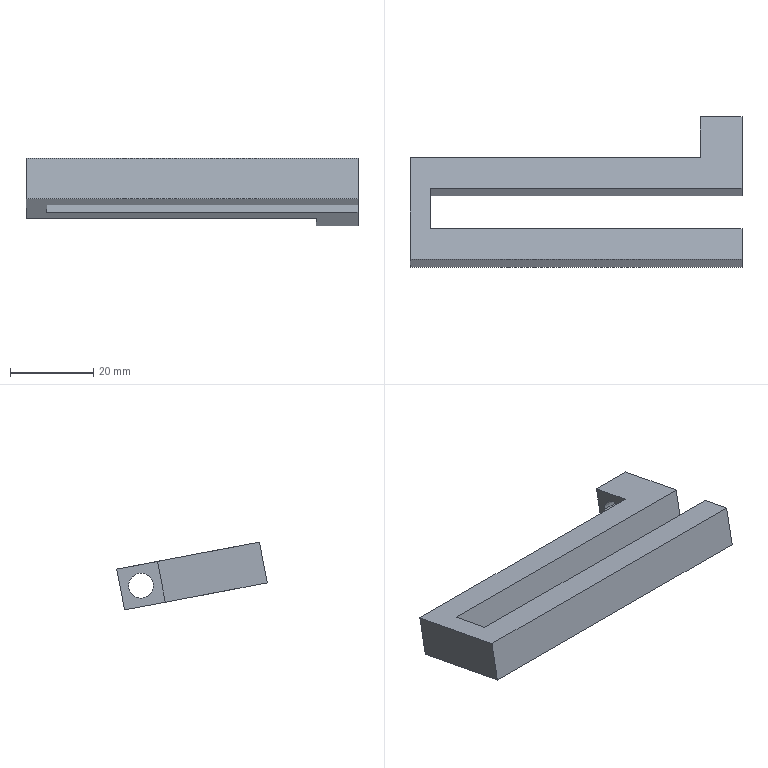Component | SolidWorks | ElectricalBoxAssembly2-1_NylonGuideBlock-1 | 1 solid | 14 faces | box 80 x 36.25 x 16.36 mm | volume 13217 mm3 | plane 12 | cylinder 2 | commonest cylinder face diameters 6 x2
build123d program:
from build123d import *

# Parameters (mm, degrees)
BOSS_EXTRUDE1_DEPTH = 10
SKETCH2_R           = 3
CUT_EXTRUDE1_DEPTH  = 83.5


with BuildPart() as part:
    # Sketch1 → Boss-Extrude1 (new body)
    with BuildSketch(Plane.XY):
        Polygon((-35.667, 17.5), (-35.667, 10), (39.333, 10), (39.333, 0), (-35.667, 0), (-35.667, -17.5), (-25.667, -17.5), (-25.667, -7.5), (44.333, -7.5), (44.333, 17.5), align=None)
    extrude(amount=BOSS_EXTRUDE1_DEPTH)

    # Sketch2 → Cut-Extrude1 (cut, through all)
    with BuildSketch(Plane.ZY.offset(35.667)):
        with Locations(Location((5, -12.5, 0), (0, 0, 270))):
            Circle(SKETCH2_R)
    extrude(amount=-CUT_EXTRUDE1_DEPTH, mode=Mode.SUBTRACT)


solid = part.part

# Placed as in the assembly
solid = solid.moved(Location((704.802, 360.896, 1985.392), (-10.755, 0, 180)))
STEP:
#1=COLOUR_RGB('',0.7922,0.8196,0.9333);
#2=FILL_AREA_STYLE_COLOUR('',#1);
#3=FILL_AREA_STYLE('',(#2));
#4=SURFACE_STYLE_FILL_AREA(#3);
#5=SURFACE_SIDE_STYLE('',(#4));
#6=SURFACE_STYLE_USAGE(.BOTH.,#5);
#7=PRESENTATION_STYLE_ASSIGNMENT((#6));
#8=CARTESIAN_POINT('',(28.759,14.613,78.289));
#9=VERTEX_POINT('',#8);
#10=CARTESIAN_POINT('',(28.759,14.845,78.245));
#11=VERTEX_POINT('',#10);
#12=CARTESIAN_POINT('',(28.759,14.729,78.267));
#13=DIRECTION('',(1.,-0.,0.));
#14=DIRECTION('',(0.,0.9824,-0.1866));
#15=AXIS2_PLACEMENT_3D('',#12,#13,#14);
#16=CIRCLE('',#15,0.1181);
#17=EDGE_CURVE('',#9,#11,#16,.T.);
#18=ORIENTED_EDGE('',*,*,#17,.F.);
#19=CARTESIAN_POINT('',(29.152,14.613,78.289));
#20=VERTEX_POINT('',#19);
#21=CARTESIAN_POINT('',(26.003,14.613,78.289));
#22=DIRECTION('',(1.,0.,0.));
#23=VECTOR('',#22,39.37);
#24=LINE('',#21,#23);
#25=EDGE_CURVE('',#9,#20,#24,.T.);
#26=ORIENTED_EDGE('',*,*,#25,.T.);
#27=CARTESIAN_POINT('',(29.152,14.845,78.245));
#28=VERTEX_POINT('',#27);
#29=CARTESIAN_POINT('',(29.152,14.729,78.267));
#30=DIRECTION('',(1.,0.,0.));
#31=DIRECTION('',(0.,0.9824,-0.1866));
#32=AXIS2_PLACEMENT_3D('',#29,#30,#31);
#33=CIRCLE('',#32,0.1181);
#34=EDGE_CURVE('',#20,#28,#33,.T.);
#35=ORIENTED_EDGE('',*,*,#34,.T.);
#36=CARTESIAN_POINT('',(26.003,14.845,78.245));
#37=DIRECTION('',(1.,0.,0.));
#38=VECTOR('',#37,39.37);
#39=LINE('',#36,#38);
#40=EDGE_CURVE('',#11,#28,#39,.T.);
#41=ORIENTED_EDGE('',*,*,#40,.F.);
#42=EDGE_LOOP('',(#18,#26,#35,#41));
#43=FACE_OUTER_BOUND('',#42,.T.);
#44=CARTESIAN_POINT('',(26.003,14.729,78.267));
#45=DIRECTION('',(1.,0.,0.));
#46=DIRECTION('',(0.,0.9824,-0.1866));
#47=AXIS2_PLACEMENT_3D('',#44,#45,#46);
#48=CYLINDRICAL_SURFACE('',#47,0.1181);
#49=ADVANCED_FACE('',(#43),#48,.F.);
#50=CARTESIAN_POINT('',(26.003,13.532,78.294));
#51=VERTEX_POINT('',#50);
#52=CARTESIAN_POINT('',(29.152,13.532,78.294));
#53=VERTEX_POINT('',#52);
#54=CARTESIAN_POINT('',(29.152,13.532,78.294));
#55=DIRECTION('',(1.,-0.,0.));
#56=VECTOR('',#55,39.37);
#57=LINE('',#54,#56);
#58=EDGE_CURVE('',#51,#53,#57,.T.);
#59=ORIENTED_EDGE('',*,*,#58,.T.);
#60=CARTESIAN_POINT('',(29.152,13.605,78.68));
#61=VERTEX_POINT('',#60);
#62=CARTESIAN_POINT('',(29.152,13.605,78.68));
#63=DIRECTION('',(0.,-0.1866,-0.9824));
#64=VECTOR('',#63,39.37);
#65=LINE('',#62,#64);
#66=EDGE_CURVE('',#61,#53,#65,.T.);
#67=ORIENTED_EDGE('',*,*,#66,.F.);
#68=CARTESIAN_POINT('',(26.003,13.605,78.68));
#69=VERTEX_POINT('',#68);
#70=CARTESIAN_POINT('',(29.152,13.605,78.68));
#71=DIRECTION('',(1.,-0.,0.));
#72=VECTOR('',#71,39.37);
#73=LINE('',#70,#72);
#74=EDGE_CURVE('',#69,#61,#73,.T.);
#75=ORIENTED_EDGE('',*,*,#74,.F.);
#76=CARTESIAN_POINT('',(26.003,13.605,78.68));
#77=DIRECTION('',(0.,-0.1866,-0.9824));
#78=VECTOR('',#77,39.37);
#79=LINE('',#76,#78);
#80=EDGE_CURVE('',#69,#51,#79,.T.);
#81=ORIENTED_EDGE('',*,*,#80,.T.);
#82=EDGE_LOOP('',(#59,#67,#75,#81));
#83=FACE_OUTER_BOUND('',#82,.T.);
#84=CARTESIAN_POINT('',(29.152,13.605,78.68));
#85=DIRECTION('',(0.,0.9824,-0.1866));
#86=DIRECTION('',(-1.,0.,-0.));
#87=AXIS2_PLACEMENT_3D('',#84,#85,#86);
#88=PLANE('',#87);
#89=ADVANCED_FACE('',(#83),#88,.F.);
#90=CARTESIAN_POINT('',(29.152,13.822,78.239));
#91=VERTEX_POINT('',#90);
#92=CARTESIAN_POINT('',(29.152,13.532,78.294));
#93=DIRECTION('',(0.,0.9824,-0.1866));
#94=VECTOR('',#93,39.37);
#95=LINE('',#92,#94);
#96=EDGE_CURVE('',#53,#91,#95,.T.);
#97=ORIENTED_EDGE('',*,*,#96,.T.);
#98=CARTESIAN_POINT('',(29.152,13.895,78.625));
#99=VERTEX_POINT('',#98);
#100=CARTESIAN_POINT('',(29.152,13.895,78.625));
#101=DIRECTION('',(0.,-0.1866,-0.9824));
#102=VECTOR('',#101,39.37);
#103=LINE('',#100,#102);
#104=EDGE_CURVE('',#99,#91,#103,.T.);
#105=ORIENTED_EDGE('',*,*,#104,.F.);
#106=CARTESIAN_POINT('',(29.152,13.605,78.68));
#107=DIRECTION('',(0.,0.9824,-0.1866));
#108=VECTOR('',#107,39.37);
#109=LINE('',#106,#108);
#110=EDGE_CURVE('',#61,#99,#109,.T.);
#111=ORIENTED_EDGE('',*,*,#110,.F.);
#112=ORIENTED_EDGE('',*,*,#66,.T.);
#113=EDGE_LOOP('',(#97,#105,#111,#112));
#114=FACE_OUTER_BOUND('',#113,.T.);
#115=CARTESIAN_POINT('',(29.152,13.605,78.68));
#116=DIRECTION('',(-1.,0.,-0.));
#117=DIRECTION('',(0.,-0.1866,-0.9824));
#118=AXIS2_PLACEMENT_3D('',#115,#116,#117);
#119=PLANE('',#118);
#120=ADVANCED_FACE('',(#114),#119,.F.);
#121=CARTESIAN_POINT('',(26.2,13.822,78.239));
#122=VERTEX_POINT('',#121);
#123=CARTESIAN_POINT('',(29.152,13.822,78.239));
#124=DIRECTION('',(-1.,0.,-0.));
#125=VECTOR('',#124,39.37);
#126=LINE('',#123,#125);
#127=EDGE_CURVE('',#91,#122,#126,.T.);
#128=ORIENTED_EDGE('',*,*,#127,.T.);
#129=CARTESIAN_POINT('',(26.2,13.895,78.625));
#130=VERTEX_POINT('',#129);
#131=CARTESIAN_POINT('',(26.2,13.895,78.625));
#132=DIRECTION('',(0.,-0.1866,-0.9824));
#133=VECTOR('',#132,39.37);
#134=LINE('',#131,#133);
#135=EDGE_CURVE('',#130,#122,#134,.T.);
#136=ORIENTED_EDGE('',*,*,#135,.F.);
#137=CARTESIAN_POINT('',(29.152,13.895,78.625));
#138=DIRECTION('',(-1.,0.,-0.));
#139=VECTOR('',#138,39.37);
#140=LINE('',#137,#139);
#141=EDGE_CURVE('',#99,#130,#140,.T.);
#142=ORIENTED_EDGE('',*,*,#141,.F.);
#143=ORIENTED_EDGE('',*,*,#104,.T.);
#144=EDGE_LOOP('',(#128,#136,#142,#143));
#145=FACE_OUTER_BOUND('',#144,.T.);
#146=CARTESIAN_POINT('',(29.152,13.895,78.625));
#147=DIRECTION('',(-0.,-0.9824,0.1866));
#148=DIRECTION('',(-0.,0.1866,0.9824));
#149=AXIS2_PLACEMENT_3D('',#146,#147,#148);
#150=PLANE('',#149);
#151=ADVANCED_FACE('',(#145),#150,.F.);
#152=CARTESIAN_POINT('',(26.2,14.209,78.165));
#153=VERTEX_POINT('',#152);
#154=CARTESIAN_POINT('',(26.2,13.822,78.239));
#155=DIRECTION('',(0.,0.9824,-0.1866));
#156=VECTOR('',#155,39.37);
#157=LINE('',#154,#156);
#158=EDGE_CURVE('',#122,#153,#157,.T.);
#159=ORIENTED_EDGE('',*,*,#158,.T.);
#160=CARTESIAN_POINT('',(26.2,14.282,78.552));
#161=VERTEX_POINT('',#160);
#162=CARTESIAN_POINT('',(26.2,14.282,78.552));
#163=DIRECTION('',(0.,-0.1866,-0.9824));
#164=VECTOR('',#163,39.37);
#165=LINE('',#162,#164);
#166=EDGE_CURVE('',#161,#153,#165,.T.);
#167=ORIENTED_EDGE('',*,*,#166,.F.);
#168=CARTESIAN_POINT('',(26.2,13.895,78.625));
#169=DIRECTION('',(0.,0.9824,-0.1866));
#170=VECTOR('',#169,39.37);
#171=LINE('',#168,#170);
#172=EDGE_CURVE('',#130,#161,#171,.T.);
#173=ORIENTED_EDGE('',*,*,#172,.F.);
#174=ORIENTED_EDGE('',*,*,#135,.T.);
#175=EDGE_LOOP('',(#159,#167,#173,#174));
#176=FACE_OUTER_BOUND('',#175,.T.);
#177=CARTESIAN_POINT('',(26.2,13.895,78.625));
#178=DIRECTION('',(-1.,0.,-0.));
#179=DIRECTION('',(-0.,-0.9824,0.1866));
#180=AXIS2_PLACEMENT_3D('',#177,#178,#179);
#181=PLANE('',#180);
#182=ADVANCED_FACE('',(#176),#181,.F.);
#183=CARTESIAN_POINT('',(29.152,14.209,78.165));
#184=VERTEX_POINT('',#183);
#185=CARTESIAN_POINT('',(26.2,14.209,78.165));
#186=DIRECTION('',(1.,-0.,0.));
#187=VECTOR('',#186,39.37);
#188=LINE('',#185,#187);
#189=EDGE_CURVE('',#153,#184,#188,.T.);
#190=ORIENTED_EDGE('',*,*,#189,.T.);
#191=CARTESIAN_POINT('',(29.152,14.282,78.552));
#192=VERTEX_POINT('',#191);
#193=CARTESIAN_POINT('',(29.152,14.282,78.552));
#194=DIRECTION('',(0.,-0.1866,-0.9824));
#195=VECTOR('',#194,39.37);
#196=LINE('',#193,#195);
#197=EDGE_CURVE('',#192,#184,#196,.T.);
#198=ORIENTED_EDGE('',*,*,#197,.F.);
#199=CARTESIAN_POINT('',(26.2,14.282,78.552));
#200=DIRECTION('',(1.,-0.,0.));
#201=VECTOR('',#200,39.37);
#202=LINE('',#199,#201);
#203=EDGE_CURVE('',#161,#192,#202,.T.);
#204=ORIENTED_EDGE('',*,*,#203,.F.);
#205=ORIENTED_EDGE('',*,*,#166,.T.);
#206=EDGE_LOOP('',(#190,#198,#204,#205));
#207=FACE_OUTER_BOUND('',#206,.T.);
#208=CARTESIAN_POINT('',(26.2,14.282,78.552));
#209=DIRECTION('',(0.,0.9824,-0.1866));
#210=DIRECTION('',(-1.,0.,-0.));
#211=AXIS2_PLACEMENT_3D('',#208,#209,#210);
#212=PLANE('',#211);
#213=ADVANCED_FACE('',(#207),#212,.F.);
#214=CARTESIAN_POINT('',(29.152,14.729,78.267));
#215=DIRECTION('',(1.,0.,0.));
#216=DIRECTION('',(0.,0.9824,-0.1866));
#217=AXIS2_PLACEMENT_3D('',#214,#215,#216);
#218=CIRCLE('',#217,0.1181);
#219=EDGE_CURVE('',#28,#20,#218,.T.);
#220=ORIENTED_EDGE('',*,*,#219,.F.);
#221=ORIENTED_EDGE('',*,*,#34,.F.);
#222=EDGE_LOOP('',(#220,#221));
#223=FACE_BOUND('',#222,.T.);
#224=CARTESIAN_POINT('',(29.152,14.885,78.036));
#225=VERTEX_POINT('',#224);
#226=CARTESIAN_POINT('',(29.152,14.209,78.165));
#227=DIRECTION('',(0.,0.9824,-0.1866));
#228=VECTOR('',#227,39.37);
#229=LINE('',#226,#228);
#230=EDGE_CURVE('',#184,#225,#229,.T.);
#231=ORIENTED_EDGE('',*,*,#230,.T.);
#232=CARTESIAN_POINT('',(29.152,14.959,78.423));
#233=VERTEX_POINT('',#232);
#234=CARTESIAN_POINT('',(29.152,14.959,78.423));
#235=DIRECTION('',(0.,-0.1866,-0.9824));
#236=VECTOR('',#235,39.37);
#237=LINE('',#234,#236);
#238=EDGE_CURVE('',#233,#225,#237,.T.);
#239=ORIENTED_EDGE('',*,*,#238,.F.);
#240=CARTESIAN_POINT('',(29.152,14.282,78.552));
#241=DIRECTION('',(0.,0.9824,-0.1866));
#242=VECTOR('',#241,39.37);
#243=LINE('',#240,#242);
#244=EDGE_CURVE('',#192,#233,#243,.T.);
#245=ORIENTED_EDGE('',*,*,#244,.F.);
#246=ORIENTED_EDGE('',*,*,#197,.T.);
#247=EDGE_LOOP('',(#231,#239,#245,#246));
#248=FACE_OUTER_BOUND('',#247,.T.);
#249=CARTESIAN_POINT('',(29.152,14.282,78.552));
#250=DIRECTION('',(-1.,-0.,-0.));
#251=DIRECTION('',(-0.,-0.9824,0.1866));
#252=AXIS2_PLACEMENT_3D('',#249,#250,#251);
#253=PLANE('',#252);
#254=ADVANCED_FACE('',(#223,#248),#253,.F.);
#255=CARTESIAN_POINT('',(28.759,14.885,78.036));
#256=VERTEX_POINT('',#255);
#257=CARTESIAN_POINT('',(29.152,14.885,78.036));
#258=DIRECTION('',(-1.,0.,-0.));
#259=VECTOR('',#258,39.37);
#260=LINE('',#257,#259);
#261=EDGE_CURVE('',#225,#256,#260,.T.);
#262=ORIENTED_EDGE('',*,*,#261,.T.);
#263=CARTESIAN_POINT('',(28.759,14.959,78.423));
#264=VERTEX_POINT('',#263);
#265=CARTESIAN_POINT('',(28.759,14.959,78.423));
#266=DIRECTION('',(0.,-0.1866,-0.9824));
#267=VECTOR('',#266,39.37);
#268=LINE('',#265,#267);
#269=EDGE_CURVE('',#264,#256,#268,.T.);
#270=ORIENTED_EDGE('',*,*,#269,.F.);
#271=CARTESIAN_POINT('',(29.152,14.959,78.423));
#272=DIRECTION('',(-1.,0.,-0.));
#273=VECTOR('',#272,39.37);
#274=LINE('',#271,#273);
#275=EDGE_CURVE('',#233,#264,#274,.T.);
#276=ORIENTED_EDGE('',*,*,#275,.F.);
#277=ORIENTED_EDGE('',*,*,#238,.T.);
#278=EDGE_LOOP('',(#262,#270,#276,#277));
#279=FACE_OUTER_BOUND('',#278,.T.);
#280=CARTESIAN_POINT('',(29.152,14.959,78.423));
#281=DIRECTION('',(-0.,-0.9824,0.1866));
#282=DIRECTION('',(-0.,0.1866,0.9824));
#283=AXIS2_PLACEMENT_3D('',#280,#281,#282);
#284=PLANE('',#283);
#285=ADVANCED_FACE('',(#279),#284,.F.);
#286=CARTESIAN_POINT('',(28.759,14.729,78.267));
#287=DIRECTION('',(1.,-0.,0.));
#288=DIRECTION('',(0.,0.9824,-0.1866));
#289=AXIS2_PLACEMENT_3D('',#286,#287,#288);
#290=CIRCLE('',#289,0.1181);
#291=EDGE_CURVE('',#11,#9,#290,.T.);
#292=ORIENTED_EDGE('',*,*,#291,.T.);
#293=ORIENTED_EDGE('',*,*,#17,.T.);
#294=EDGE_LOOP('',(#292,#293));
#295=FACE_BOUND('',#294,.T.);
#296=CARTESIAN_POINT('',(28.759,14.499,78.11));
#297=VERTEX_POINT('',#296);
#298=CARTESIAN_POINT('',(28.759,14.499,78.11));
#299=DIRECTION('',(-0.,-0.9824,0.1866));
#300=VECTOR('',#299,39.37);
#301=LINE('',#298,#300);
#302=EDGE_CURVE('',#256,#297,#301,.T.);
#303=ORIENTED_EDGE('',*,*,#302,.T.);
#304=CARTESIAN_POINT('',(28.759,14.572,78.497));
#305=VERTEX_POINT('',#304);
#306=CARTESIAN_POINT('',(28.759,14.572,78.497));
#307=DIRECTION('',(0.,-0.1866,-0.9824));
#308=VECTOR('',#307,39.37);
#309=LINE('',#306,#308);
#310=EDGE_CURVE('',#305,#297,#309,.T.);
#311=ORIENTED_EDGE('',*,*,#310,.F.);
#312=CARTESIAN_POINT('',(28.759,14.572,78.497));
#313=DIRECTION('',(-0.,-0.9824,0.1866));
#314=VECTOR('',#313,39.37);
#315=LINE('',#312,#314);
#316=EDGE_CURVE('',#264,#305,#315,.T.);
#317=ORIENTED_EDGE('',*,*,#316,.F.);
#318=ORIENTED_EDGE('',*,*,#269,.T.);
#319=EDGE_LOOP('',(#303,#311,#317,#318));
#320=FACE_OUTER_BOUND('',#319,.T.);
#321=CARTESIAN_POINT('',(28.759,14.572,78.497));
#322=DIRECTION('',(1.,-0.,0.));
#323=DIRECTION('',(0.,0.9824,-0.1866));
#324=AXIS2_PLACEMENT_3D('',#321,#322,#323);
#325=PLANE('',#324);
#326=ADVANCED_FACE('',(#295,#320),#325,.F.);
#327=CARTESIAN_POINT('',(26.003,14.499,78.11));
#328=VERTEX_POINT('',#327);
#329=CARTESIAN_POINT('',(26.003,14.499,78.11));
#330=DIRECTION('',(-1.,0.,-0.));
#331=VECTOR('',#330,39.37);
#332=LINE('',#329,#331);
#333=EDGE_CURVE('',#297,#328,#332,.T.);
#334=ORIENTED_EDGE('',*,*,#333,.T.);
#335=CARTESIAN_POINT('',(26.003,14.572,78.497));
#336=VERTEX_POINT('',#335);
#337=CARTESIAN_POINT('',(26.003,14.572,78.497));
#338=DIRECTION('',(0.,-0.1866,-0.9824));
#339=VECTOR('',#338,39.37);
#340=LINE('',#337,#339);
#341=EDGE_CURVE('',#336,#328,#340,.T.);
#342=ORIENTED_EDGE('',*,*,#341,.F.);
#343=CARTESIAN_POINT('',(26.003,14.572,78.497));
#344=DIRECTION('',(-1.,0.,-0.));
#345=VECTOR('',#344,39.37);
#346=LINE('',#343,#345);
#347=EDGE_CURVE('',#305,#336,#346,.T.);
#348=ORIENTED_EDGE('',*,*,#347,.F.);
#349=ORIENTED_EDGE('',*,*,#310,.T.);
#350=EDGE_LOOP('',(#334,#342,#348,#349));
#351=FACE_OUTER_BOUND('',#350,.T.);
#352=CARTESIAN_POINT('',(26.003,14.572,78.497));
#353=DIRECTION('',(-0.,-0.9824,0.1866));
#354=DIRECTION('',(1.,-0.,0.));
#355=AXIS2_PLACEMENT_3D('',#352,#353,#354);
#356=PLANE('',#355);
#357=ADVANCED_FACE('',(#351),#356,.F.);
#358=CARTESIAN_POINT('',(26.003,13.532,78.294));
#359=DIRECTION('',(-0.,-0.9824,0.1866));
#360=VECTOR('',#359,39.37);
#361=LINE('',#358,#360);
#362=EDGE_CURVE('',#328,#51,#361,.T.);
#363=ORIENTED_EDGE('',*,*,#362,.T.);
#364=ORIENTED_EDGE('',*,*,#80,.F.);
#365=CARTESIAN_POINT('',(26.003,13.605,78.68));
#366=DIRECTION('',(-0.,-0.9824,0.1866));
#367=VECTOR('',#366,39.37);
#368=LINE('',#365,#367);
#369=EDGE_CURVE('',#336,#69,#368,.T.);
#370=ORIENTED_EDGE('',*,*,#369,.F.);
#371=ORIENTED_EDGE('',*,*,#341,.T.);
#372=EDGE_LOOP('',(#363,#364,#370,#371));
#373=FACE_OUTER_BOUND('',#372,.T.);
#374=CARTESIAN_POINT('',(26.003,13.605,78.68));
#375=DIRECTION('',(1.,-0.,0.));
#376=DIRECTION('',(-0.,0.1866,0.9824));
#377=AXIS2_PLACEMENT_3D('',#374,#375,#376);
#378=PLANE('',#377);
#379=ADVANCED_FACE('',(#373),#378,.F.);
#380=ORIENTED_EDGE('',*,*,#74,.T.);
#381=ORIENTED_EDGE('',*,*,#110,.T.);
#382=ORIENTED_EDGE('',*,*,#141,.T.);
#383=ORIENTED_EDGE('',*,*,#172,.T.);
#384=ORIENTED_EDGE('',*,*,#203,.T.);
#385=ORIENTED_EDGE('',*,*,#244,.T.);
#386=ORIENTED_EDGE('',*,*,#275,.T.);
#387=ORIENTED_EDGE('',*,*,#316,.T.);
#388=ORIENTED_EDGE('',*,*,#347,.T.);
#389=ORIENTED_EDGE('',*,*,#369,.T.);
#390=EDGE_LOOP('',(#380,#381,#382,#383,#384,#385,#386,#387,#388,#389));
#391=FACE_OUTER_BOUND('',#390,.T.);
#392=CARTESIAN_POINT('',(27.748,14.282,78.552));
#393=DIRECTION('',(0.,-0.1866,-0.9824));
#394=DIRECTION('',(1.,-0.,0.));
#395=AXIS2_PLACEMENT_3D('',#392,#393,#394);
#396=PLANE('',#395);
#397=ADVANCED_FACE('',(#391),#396,.F.);
#398=ORIENTED_EDGE('',*,*,#58,.F.);
#399=ORIENTED_EDGE('',*,*,#362,.F.);
#400=ORIENTED_EDGE('',*,*,#333,.F.);
#401=ORIENTED_EDGE('',*,*,#302,.F.);
#402=ORIENTED_EDGE('',*,*,#261,.F.);
#403=ORIENTED_EDGE('',*,*,#230,.F.);
#404=ORIENTED_EDGE('',*,*,#189,.F.);
#405=ORIENTED_EDGE('',*,*,#158,.F.);
#406=ORIENTED_EDGE('',*,*,#127,.F.);
#407=ORIENTED_EDGE('',*,*,#96,.F.);
#408=EDGE_LOOP('',(#398,#399,#400,#401,#402,#403,#404,#405,#406,#407));
#409=FACE_OUTER_BOUND('',#408,.T.);
#410=CARTESIAN_POINT('',(27.748,14.209,78.165));
#411=DIRECTION('',(0.,-0.1866,-0.9824));
#412=DIRECTION('',(1.,-0.,0.));
#413=AXIS2_PLACEMENT_3D('',#410,#411,#412);
#414=PLANE('',#413);
#415=ADVANCED_FACE('',(#409),#414,.T.);
#416=ORIENTED_EDGE('',*,*,#25,.F.);
#417=ORIENTED_EDGE('',*,*,#291,.F.);
#418=ORIENTED_EDGE('',*,*,#40,.T.);
#419=ORIENTED_EDGE('',*,*,#219,.T.);
#420=EDGE_LOOP('',(#416,#417,#418,#419));
#421=FACE_OUTER_BOUND('',#420,.T.);
#422=CARTESIAN_POINT('',(26.003,14.729,78.267));
#423=DIRECTION('',(1.,0.,0.));
#424=DIRECTION('',(0.,0.9824,-0.1866));
#425=AXIS2_PLACEMENT_3D('',#422,#423,#424);
#426=CYLINDRICAL_SURFACE('',#425,0.1181);
#427=ADVANCED_FACE('',(#421),#426,.F.);
#428=CLOSED_SHELL('',(#49,#89,#120,#151,#182,#213,#254,#285,#326,#357,#379,#397,#415,#427));
#429=MANIFOLD_SOLID_BREP('',#428);
#430=STYLED_ITEM('',(#7),#429);
#431=PRESENTATION_LAYER_ASSIGNMENT('','',(#430));
#432=(LENGTH_UNIT()NAMED_UNIT(*)SI_UNIT($,.METRE.));
#433=LENGTH_MEASURE_WITH_UNIT(LENGTH_MEASURE(0.0254),#432);
#434=DIMENSIONAL_EXPONENTS(1.,0.,0.,0.,0.,0.,0.);
#435=(CONVERSION_BASED_UNIT('',#433)LENGTH_UNIT()NAMED_UNIT(#434));
#436=UNCERTAINTY_MEASURE_WITH_UNIT(LENGTH_MEASURE(0.00001),#435,'','');
#437=(NAMED_UNIT(*)PLANE_ANGLE_UNIT()SI_UNIT($,.RADIAN.));
#438=(NAMED_UNIT(*)SI_UNIT($,.STERADIAN.)SOLID_ANGLE_UNIT());
#439=(GEOMETRIC_REPRESENTATION_CONTEXT(3)GLOBAL_UNCERTAINTY_ASSIGNED_CONTEXT((#436))GLOBAL_UNIT_ASSIGNED_CONTEXT((#435,#437,#438))REPRESENTATION_CONTEXT('',''));
#440=MECHANICAL_DESIGN_GEOMETRIC_PRESENTATION_REPRESENTATION('',(#430),#439);
#441=CARTESIAN_POINT('',(0.,0.,0.));
#442=DIRECTION('',(0.,0.,1.));
#443=DIRECTION('',(1.,0.,0.));
#444=AXIS2_PLACEMENT_3D('',#441,#442,#443);
#445=(LENGTH_UNIT()NAMED_UNIT(*)SI_UNIT($,.METRE.));
#446=LENGTH_MEASURE_WITH_UNIT(LENGTH_MEASURE(0.0254),#445);
#447=DIMENSIONAL_EXPONENTS(1.,0.,0.,0.,0.,0.,0.);
#448=(CONVERSION_BASED_UNIT('',#446)LENGTH_UNIT()NAMED_UNIT(#447));
#449=UNCERTAINTY_MEASURE_WITH_UNIT(LENGTH_MEASURE(0.00001),#448,'','');
#450=(NAMED_UNIT(*)PLANE_ANGLE_UNIT()SI_UNIT($,.RADIAN.));
#451=(NAMED_UNIT(*)SI_UNIT($,.STERADIAN.)SOLID_ANGLE_UNIT());
#452=(GEOMETRIC_REPRESENTATION_CONTEXT(3)GLOBAL_UNCERTAINTY_ASSIGNED_CONTEXT((#449))GLOBAL_UNIT_ASSIGNED_CONTEXT((#448,#450,#451))REPRESENTATION_CONTEXT('',''));
#453=ADVANCED_BREP_SHAPE_REPRESENTATION('',(#429,#444),#452);